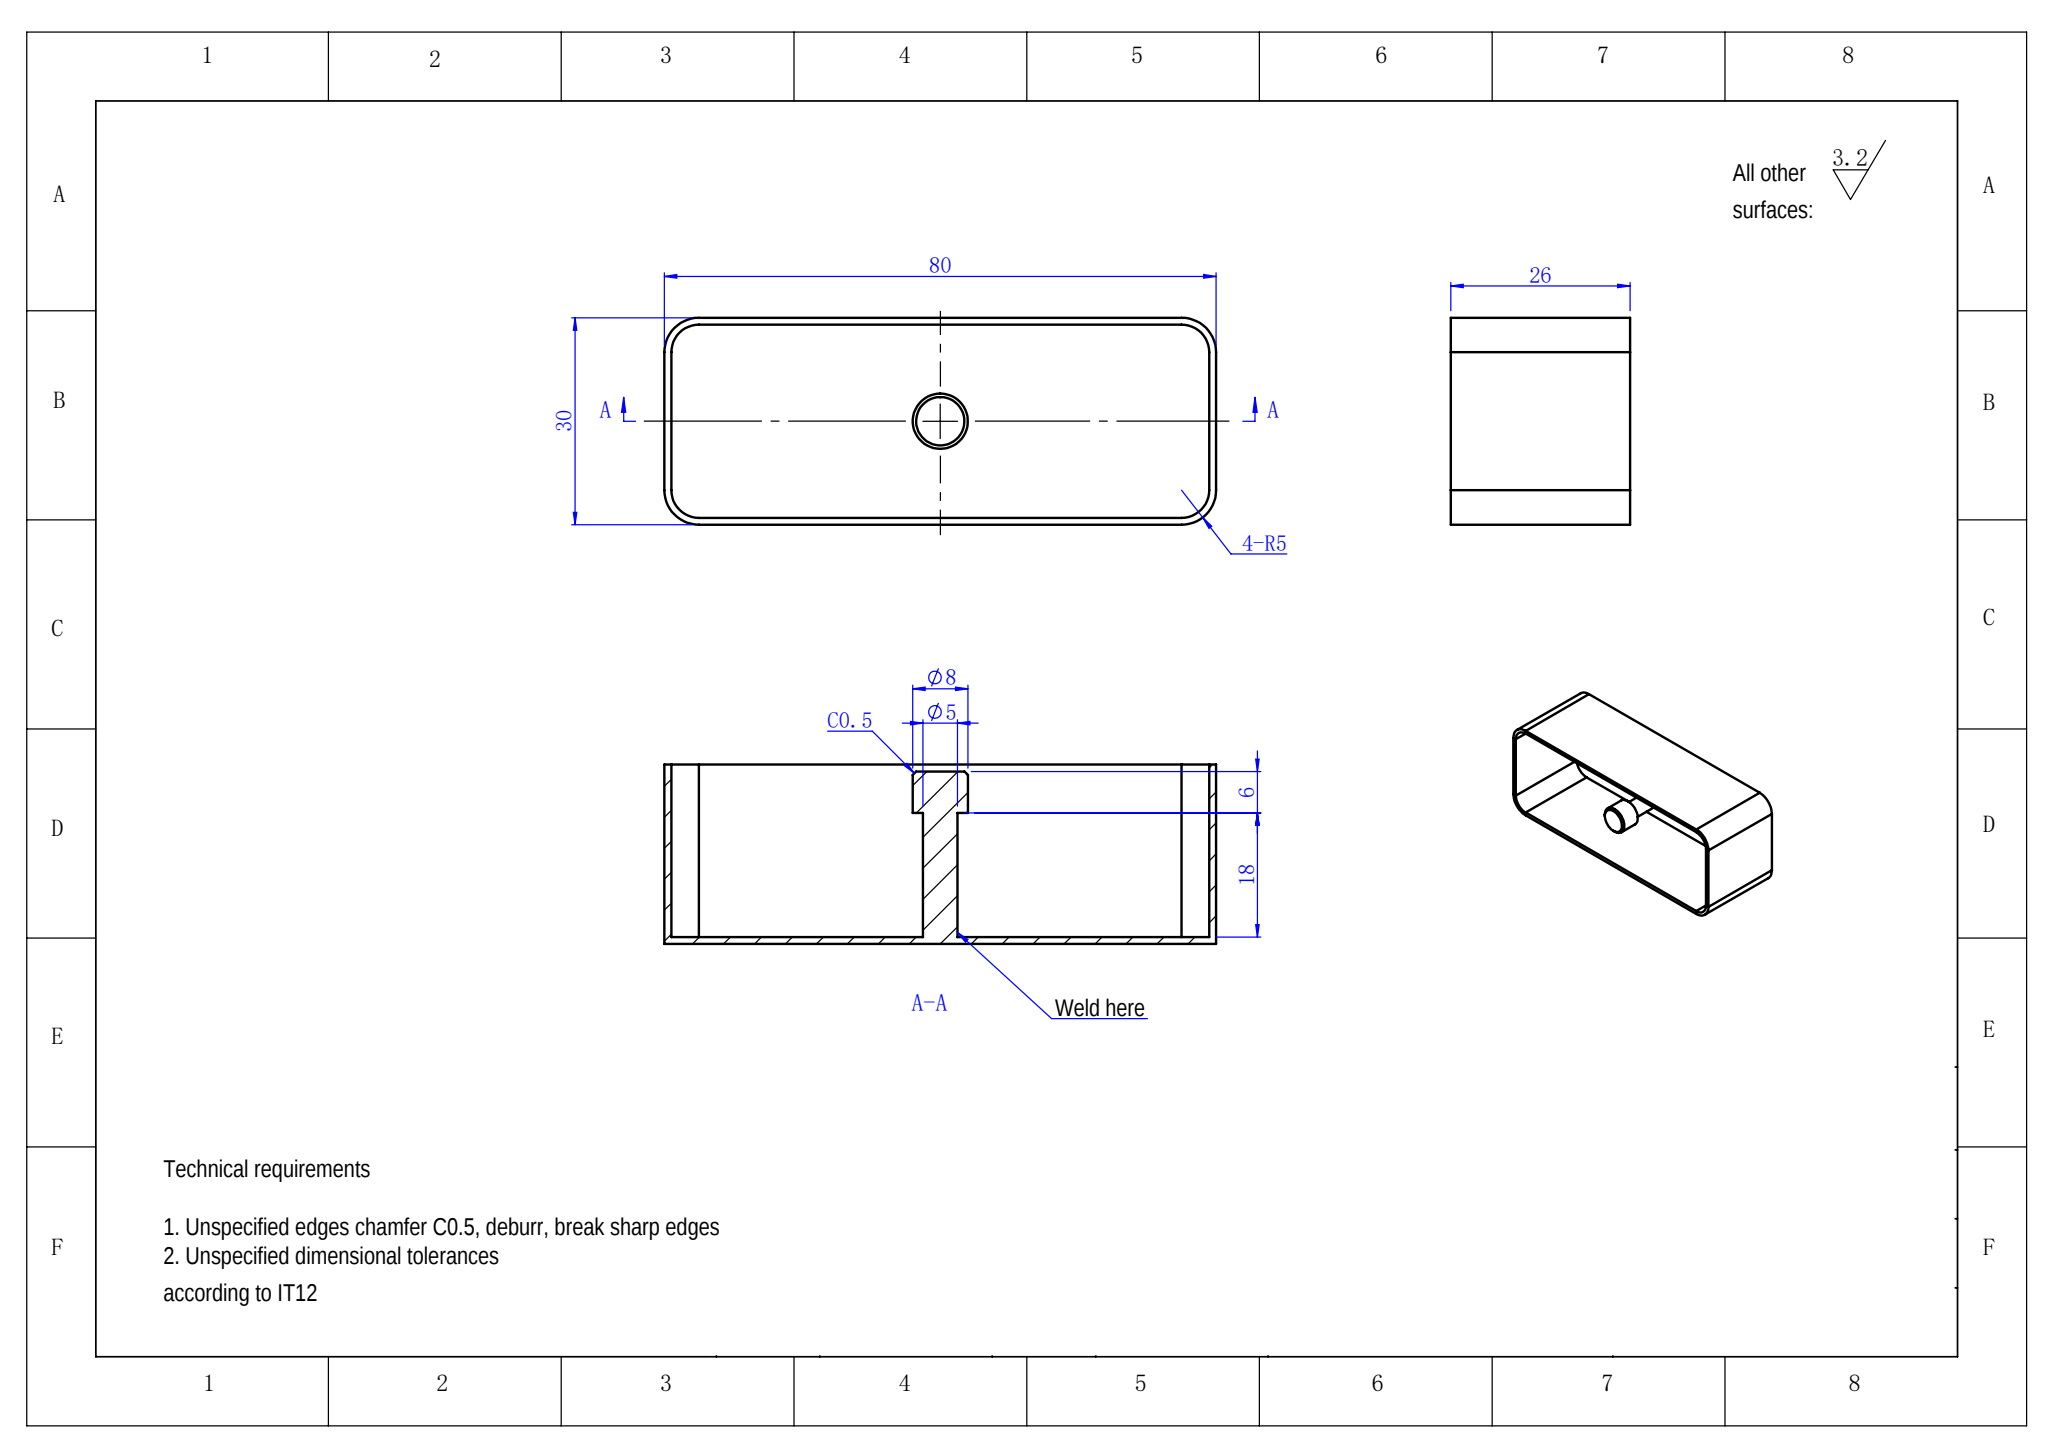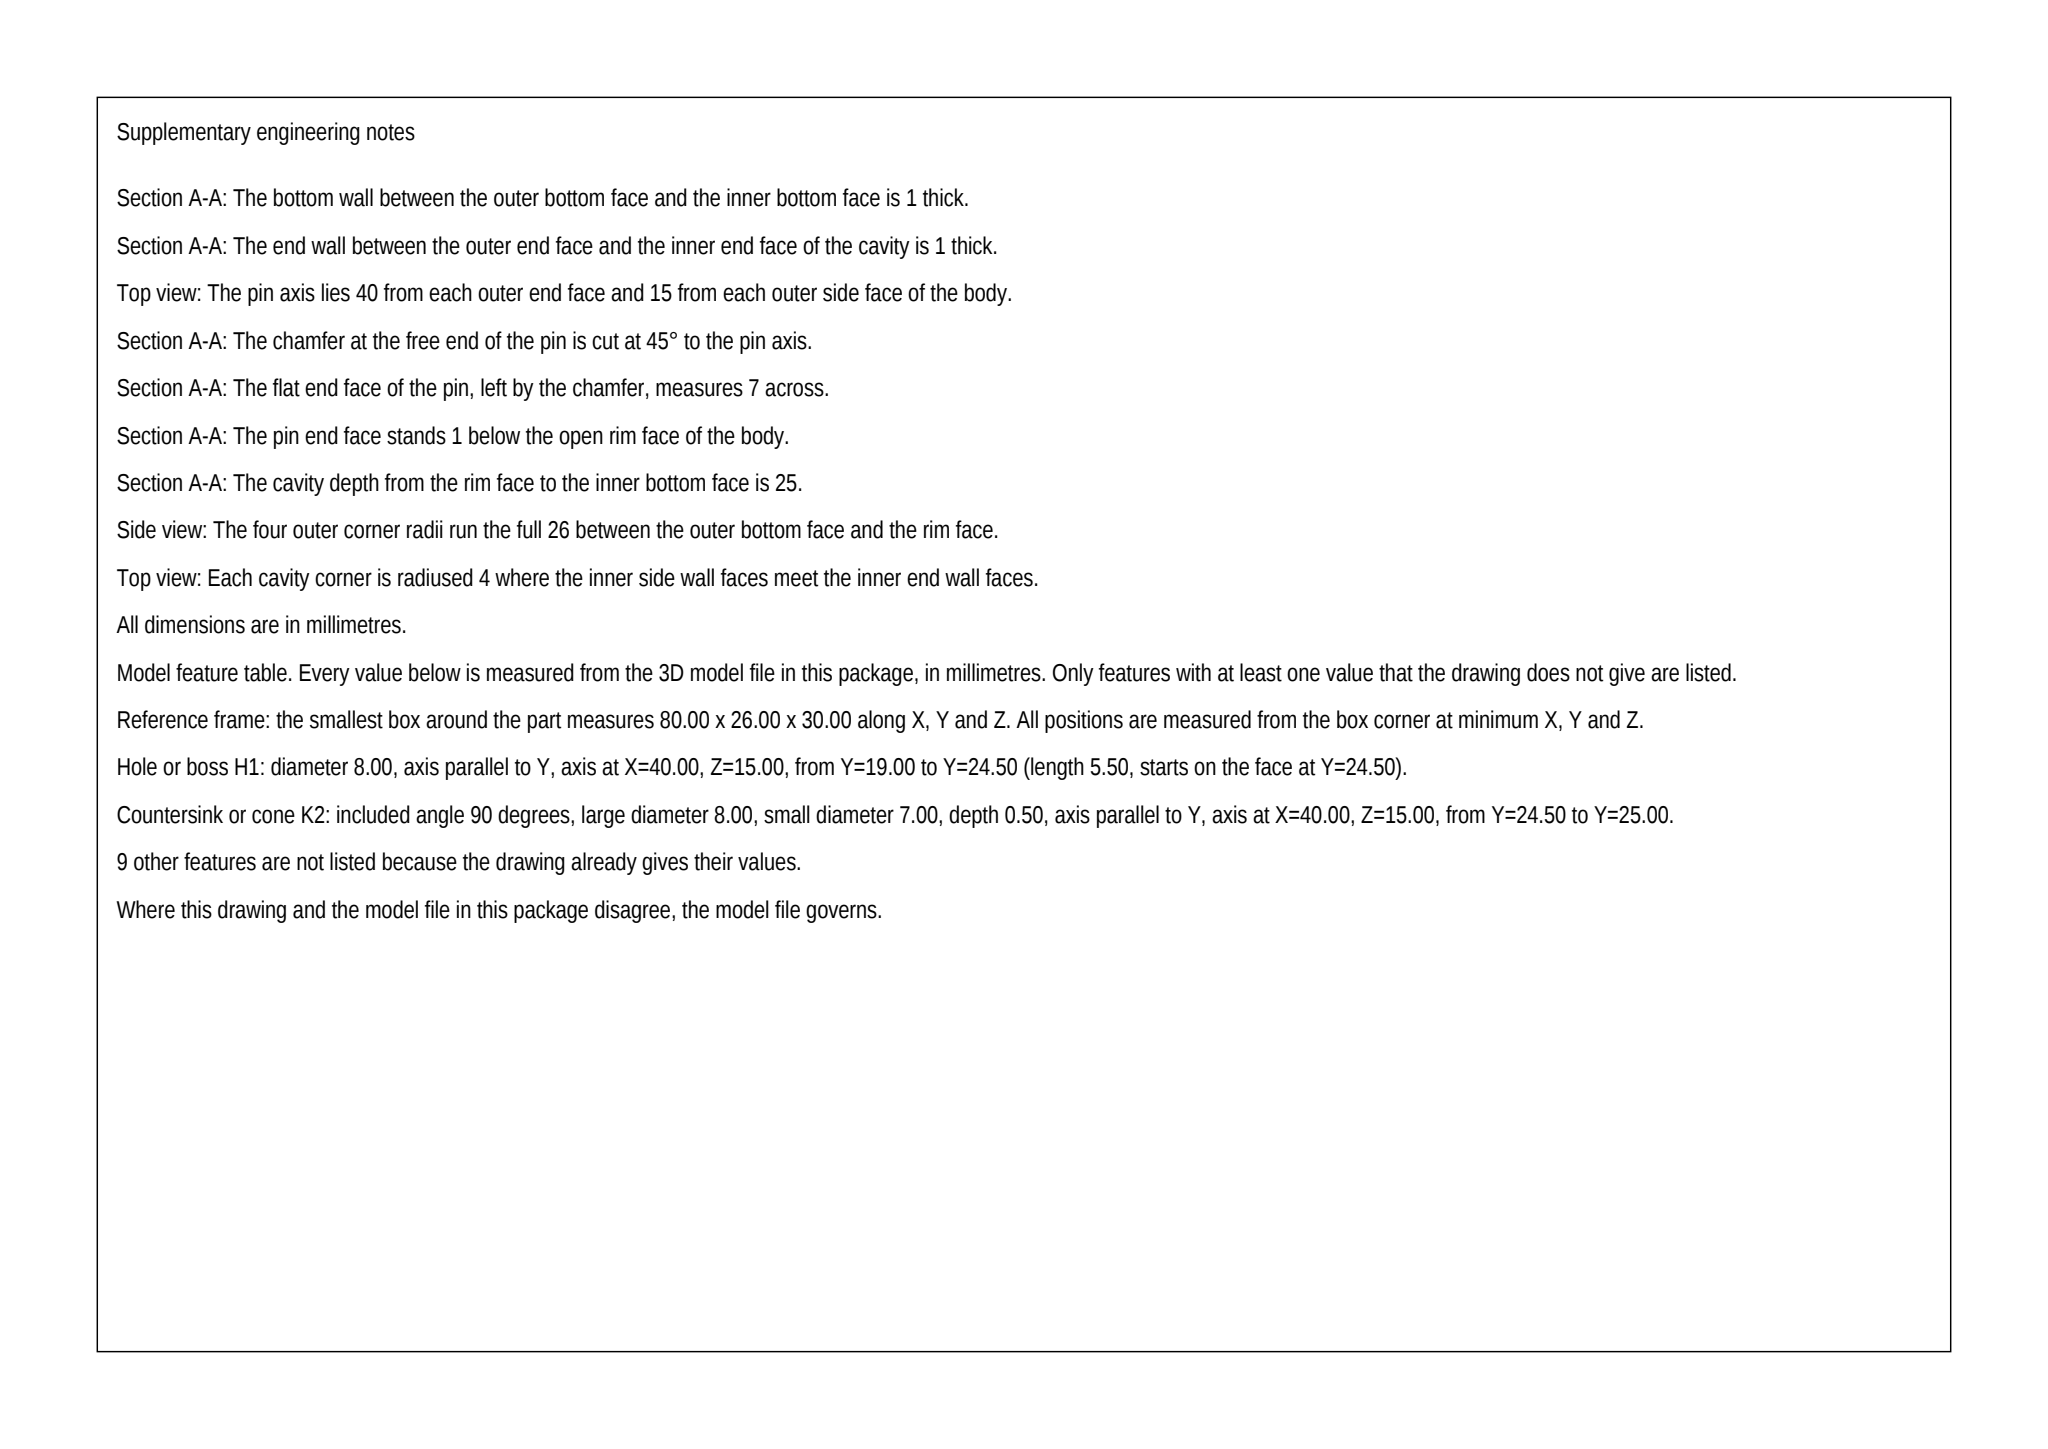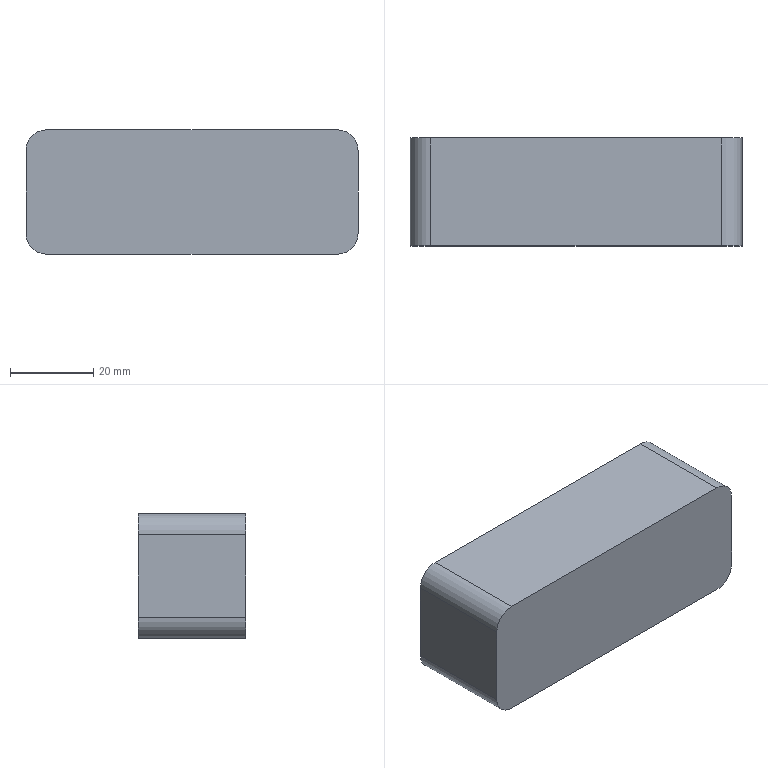Part | SolidWorks | mm | 1 solid | 27 faces | box 80 x 26 x 30 mm | volume 8237 mm3 | plane 13 | cylinder 12 | cone 2 | commonest cylinder face diameters 8 x6 10 x4 5 x2
build123d program:
from build123d import *

# Parameters (mm, degrees)
BOSS_EXTRUDE1_DEPTH = 26
SHELL1_T            = -1
CHAMFER1_SIZE       = 0.5


with BuildPart() as part:
    # Sketch1 → Boss-Extrude1 (new body)
    with BuildSketch(Plane(origin=(0, 0, 0), x_dir=(1, 0, 0), z_dir=(0, 1, 0))):
        with BuildLine():
            Line((-35, 15), (35, 15))
            ThreePointArc((35, 15), (38.536, 13.536), (40, 10))
            Line((40, 10), (40, -10))
            ThreePointArc((40, -10), (38.536, -13.536), (35, -15))
            Line((35, -15), (-35, -15))
            ThreePointArc((-35, -15), (-38.536, -13.536), (-40, -10))
            Line((-40, -10), (-40, 10))
            ThreePointArc((-40, 10), (-38.536, 13.536), (-35, 15))
        make_face()
    extrude(amount=BOSS_EXTRUDE1_DEPTH)

    # Shell1
    shell1_openings = [part.faces().sort_by_distance(p)[0] for p in [
        (0, 26, 0),
    ]]
    offset(amount=SHELL1_T, openings=shell1_openings, kind=Kind.INTERSECTION)

    # Sketch3 → Revolve1 (revolve)
    with BuildSketch(Plane.XY, mode=Mode.PRIVATE) as revolve1_sk:
        Polygon((0, 0), (-2.5, 0), (-2.5, 19), (-4, 19), (-4, 25), (0, 25), align=None)
    revolve(revolve1_sk.sketch.rotate(Axis((0, 0, 0), (0, 1, 0)), 270), axis=Axis((0, 0, 0), (0, 1, 0)))

    # Chamfer1
    chamfer1_edges = [part.edges().sort_by_distance(p)[0] for p in [
        (0, 25, 4),
    ]]
    chamfer(chamfer1_edges, length=CHAMFER1_SIZE)


solid = part.part
STEP:
#1=CARTESIAN_POINT('',(0.,25.,3.5));
#2=VERTEX_POINT('',#1);
#3=CARTESIAN_POINT('',(0.,25.,-3.5));
#4=VERTEX_POINT('',#3);
#5=CARTESIAN_POINT('',(0.,25.,0.));
#6=DIRECTION('',(0.,1.,0.));
#7=DIRECTION('',(0.,0.,-1.));
#8=AXIS2_PLACEMENT_3D('',#5,#6,#7);
#9=CIRCLE('',#8,3.5);
#10=EDGE_CURVE('',#2,#4,#9,.T.);
#11=ORIENTED_EDGE('',*,*,#10,.F.);
#12=CARTESIAN_POINT('',(0.,24.5,4.));
#13=VERTEX_POINT('',#12);
#14=CARTESIAN_POINT('',(0.,24.5,4.));
#15=DIRECTION('',(0.,-0.7071,0.7071));
#16=VECTOR('',#15,1000.);
#17=LINE('',#14,#16);
#18=EDGE_CURVE('',#2,#13,#17,.T.);
#19=ORIENTED_EDGE('',*,*,#18,.T.);
#20=CARTESIAN_POINT('',(0.,24.5,-4.));
#21=VERTEX_POINT('',#20);
#22=CARTESIAN_POINT('',(0.,24.5,0.));
#23=DIRECTION('',(0.,-1.,0.));
#24=DIRECTION('',(0.,0.,-1.));
#25=AXIS2_PLACEMENT_3D('',#22,#23,#24);
#26=CIRCLE('',#25,4.);
#27=EDGE_CURVE('',#21,#13,#26,.T.);
#28=ORIENTED_EDGE('',*,*,#27,.F.);
#29=CARTESIAN_POINT('',(0.,24.5,-4.));
#30=DIRECTION('',(0.,-0.7071,-0.7071));
#31=VECTOR('',#30,1000.);
#32=LINE('',#29,#31);
#33=EDGE_CURVE('',#4,#21,#32,.T.);
#34=ORIENTED_EDGE('',*,*,#33,.F.);
#35=EDGE_LOOP('',(#11,#19,#28,#34));
#36=FACE_OUTER_BOUND('',#35,.T.);
#37=CARTESIAN_POINT('',(0.,24.5,0.));
#38=DIRECTION('',(0.,-1.,0.));
#39=DIRECTION('',(0.,0.,-1.));
#40=AXIS2_PLACEMENT_3D('',#37,#38,#39);
#41=CONICAL_SURFACE('',#40,4.,0.7854);
#42=ADVANCED_FACE('',(#36),#41,.T.);
#43=ORIENTED_EDGE('',*,*,#27,.T.);
#44=CARTESIAN_POINT('',(0.,19.,4.));
#45=VERTEX_POINT('',#44);
#46=CARTESIAN_POINT('',(0.,0.,4.));
#47=DIRECTION('',(0.,-1.,0.));
#48=VECTOR('',#47,1000.);
#49=LINE('',#46,#48);
#50=EDGE_CURVE('',#13,#45,#49,.T.);
#51=ORIENTED_EDGE('',*,*,#50,.T.);
#52=CARTESIAN_POINT('',(0.,19.,-4.));
#53=VERTEX_POINT('',#52);
#54=CARTESIAN_POINT('',(0.,19.,0.));
#55=DIRECTION('',(0.,-1.,0.));
#56=DIRECTION('',(0.,0.,-1.));
#57=AXIS2_PLACEMENT_3D('',#54,#55,#56);
#58=CIRCLE('',#57,4.);
#59=EDGE_CURVE('',#53,#45,#58,.T.);
#60=ORIENTED_EDGE('',*,*,#59,.F.);
#61=CARTESIAN_POINT('',(0.,0.,-4.));
#62=DIRECTION('',(0.,-1.,0.));
#63=VECTOR('',#62,1000.);
#64=LINE('',#61,#63);
#65=EDGE_CURVE('',#21,#53,#64,.T.);
#66=ORIENTED_EDGE('',*,*,#65,.F.);
#67=EDGE_LOOP('',(#43,#51,#60,#66));
#68=FACE_OUTER_BOUND('',#67,.T.);
#69=CARTESIAN_POINT('',(0.,0.,0.));
#70=DIRECTION('',(0.,-1.,0.));
#71=DIRECTION('',(0.,0.,-1.));
#72=AXIS2_PLACEMENT_3D('',#69,#70,#71);
#73=CYLINDRICAL_SURFACE('',#72,4.);
#74=ADVANCED_FACE('',(#68),#73,.T.);
#75=CARTESIAN_POINT('',(0.,19.,-2.5));
#76=VERTEX_POINT('',#75);
#77=CARTESIAN_POINT('',(0.,19.,2.5));
#78=VERTEX_POINT('',#77);
#79=CARTESIAN_POINT('',(0.,19.,0.));
#80=DIRECTION('',(0.,-1.,0.));
#81=DIRECTION('',(0.,0.,-1.));
#82=AXIS2_PLACEMENT_3D('',#79,#80,#81);
#83=CIRCLE('',#82,2.5);
#84=EDGE_CURVE('',#76,#78,#83,.T.);
#85=ORIENTED_EDGE('',*,*,#84,.T.);
#86=CARTESIAN_POINT('',(0.,1.,2.5));
#87=VERTEX_POINT('',#86);
#88=CARTESIAN_POINT('',(0.,0.,2.5));
#89=DIRECTION('',(0.,-1.,0.));
#90=VECTOR('',#89,1000.);
#91=LINE('',#88,#90);
#92=EDGE_CURVE('',#78,#87,#91,.T.);
#93=ORIENTED_EDGE('',*,*,#92,.T.);
#94=CARTESIAN_POINT('',(0.,1.,-2.5));
#95=VERTEX_POINT('',#94);
#96=CARTESIAN_POINT('',(0.,1.,0.));
#97=DIRECTION('',(0.,-1.,0.));
#98=DIRECTION('',(0.,0.,1.));
#99=AXIS2_PLACEMENT_3D('',#96,#97,#98);
#100=CIRCLE('',#99,2.5);
#101=EDGE_CURVE('',#95,#87,#100,.T.);
#102=ORIENTED_EDGE('',*,*,#101,.F.);
#103=CARTESIAN_POINT('',(0.,0.,-2.5));
#104=DIRECTION('',(0.,-1.,0.));
#105=VECTOR('',#104,1000.);
#106=LINE('',#103,#105);
#107=EDGE_CURVE('',#76,#95,#106,.T.);
#108=ORIENTED_EDGE('',*,*,#107,.F.);
#109=EDGE_LOOP('',(#85,#93,#102,#108));
#110=FACE_OUTER_BOUND('',#109,.T.);
#111=CARTESIAN_POINT('',(0.,0.,0.));
#112=DIRECTION('',(0.,-1.,0.));
#113=DIRECTION('',(0.,0.,-1.));
#114=AXIS2_PLACEMENT_3D('',#111,#112,#113);
#115=CYLINDRICAL_SURFACE('',#114,2.5);
#116=ADVANCED_FACE('',(#110),#115,.T.);
#117=CARTESIAN_POINT('',(35.,0.,15.));
#118=VERTEX_POINT('',#117);
#119=CARTESIAN_POINT('',(40.,0.,10.));
#120=VERTEX_POINT('',#119);
#121=CARTESIAN_POINT('',(35.,0.,10.));
#122=DIRECTION('',(0.,1.,0.));
#123=DIRECTION('',(0.,0.,1.));
#124=AXIS2_PLACEMENT_3D('',#121,#122,#123);
#125=CIRCLE('',#124,5.);
#126=EDGE_CURVE('',#118,#120,#125,.T.);
#127=ORIENTED_EDGE('',*,*,#126,.T.);
#128=CARTESIAN_POINT('',(40.,26.,10.));
#129=VERTEX_POINT('',#128);
#130=CARTESIAN_POINT('',(40.,26.,10.));
#131=DIRECTION('',(0.,-1.,0.));
#132=VECTOR('',#131,1000.);
#133=LINE('',#130,#132);
#134=EDGE_CURVE('',#129,#120,#133,.T.);
#135=ORIENTED_EDGE('',*,*,#134,.F.);
#136=CARTESIAN_POINT('',(35.,26.,15.));
#137=VERTEX_POINT('',#136);
#138=CARTESIAN_POINT('',(35.,26.,10.));
#139=DIRECTION('',(0.,1.,0.));
#140=DIRECTION('',(0.,0.,1.));
#141=AXIS2_PLACEMENT_3D('',#138,#139,#140);
#142=CIRCLE('',#141,5.);
#143=EDGE_CURVE('',#137,#129,#142,.T.);
#144=ORIENTED_EDGE('',*,*,#143,.F.);
#145=CARTESIAN_POINT('',(35.,26.,15.));
#146=DIRECTION('',(0.,-1.,0.));
#147=VECTOR('',#146,1000.);
#148=LINE('',#145,#147);
#149=EDGE_CURVE('',#137,#118,#148,.T.);
#150=ORIENTED_EDGE('',*,*,#149,.T.);
#151=EDGE_LOOP('',(#127,#135,#144,#150));
#152=FACE_OUTER_BOUND('',#151,.T.);
#153=CARTESIAN_POINT('',(35.,26.,10.));
#154=DIRECTION('',(0.,-1.,0.));
#155=DIRECTION('',(0.,0.,-1.));
#156=AXIS2_PLACEMENT_3D('',#153,#154,#155);
#157=CYLINDRICAL_SURFACE('',#156,5.);
#158=ADVANCED_FACE('',(#152),#157,.T.);
#159=CARTESIAN_POINT('',(40.,0.,-10.));
#160=VERTEX_POINT('',#159);
#161=CARTESIAN_POINT('',(40.,0.,-10.));
#162=DIRECTION('',(0.,0.,-1.));
#163=VECTOR('',#162,1000.);
#164=LINE('',#161,#163);
#165=EDGE_CURVE('',#120,#160,#164,.T.);
#166=ORIENTED_EDGE('',*,*,#165,.T.);
#167=CARTESIAN_POINT('',(40.,26.,-10.));
#168=VERTEX_POINT('',#167);
#169=CARTESIAN_POINT('',(40.,26.,-10.));
#170=DIRECTION('',(0.,-1.,0.));
#171=VECTOR('',#170,1000.);
#172=LINE('',#169,#171);
#173=EDGE_CURVE('',#168,#160,#172,.T.);
#174=ORIENTED_EDGE('',*,*,#173,.F.);
#175=CARTESIAN_POINT('',(40.,26.,-10.));
#176=DIRECTION('',(0.,0.,-1.));
#177=VECTOR('',#176,1000.);
#178=LINE('',#175,#177);
#179=EDGE_CURVE('',#129,#168,#178,.T.);
#180=ORIENTED_EDGE('',*,*,#179,.F.);
#181=ORIENTED_EDGE('',*,*,#134,.T.);
#182=EDGE_LOOP('',(#166,#174,#180,#181));
#183=FACE_OUTER_BOUND('',#182,.T.);
#184=CARTESIAN_POINT('',(40.,26.,-10.));
#185=DIRECTION('',(-1.,0.,0.));
#186=DIRECTION('',(0.,0.,1.));
#187=AXIS2_PLACEMENT_3D('',#184,#185,#186);
#188=PLANE('',#187);
#189=ADVANCED_FACE('',(#183),#188,.F.);
#190=CARTESIAN_POINT('',(35.,0.,-15.));
#191=VERTEX_POINT('',#190);
#192=CARTESIAN_POINT('',(35.,0.,-10.));
#193=DIRECTION('',(0.,1.,0.));
#194=DIRECTION('',(0.,0.,1.));
#195=AXIS2_PLACEMENT_3D('',#192,#193,#194);
#196=CIRCLE('',#195,5.);
#197=EDGE_CURVE('',#160,#191,#196,.T.);
#198=ORIENTED_EDGE('',*,*,#197,.T.);
#199=CARTESIAN_POINT('',(35.,26.,-15.));
#200=VERTEX_POINT('',#199);
#201=CARTESIAN_POINT('',(35.,26.,-15.));
#202=DIRECTION('',(0.,-1.,0.));
#203=VECTOR('',#202,1000.);
#204=LINE('',#201,#203);
#205=EDGE_CURVE('',#200,#191,#204,.T.);
#206=ORIENTED_EDGE('',*,*,#205,.F.);
#207=CARTESIAN_POINT('',(35.,26.,-10.));
#208=DIRECTION('',(0.,1.,0.));
#209=DIRECTION('',(0.,0.,1.));
#210=AXIS2_PLACEMENT_3D('',#207,#208,#209);
#211=CIRCLE('',#210,5.);
#212=EDGE_CURVE('',#168,#200,#211,.T.);
#213=ORIENTED_EDGE('',*,*,#212,.F.);
#214=ORIENTED_EDGE('',*,*,#173,.T.);
#215=EDGE_LOOP('',(#198,#206,#213,#214));
#216=FACE_OUTER_BOUND('',#215,.T.);
#217=CARTESIAN_POINT('',(35.,26.,-10.));
#218=DIRECTION('',(0.,-1.,0.));
#219=DIRECTION('',(0.,0.,-1.));
#220=AXIS2_PLACEMENT_3D('',#217,#218,#219);
#221=CYLINDRICAL_SURFACE('',#220,5.);
#222=ADVANCED_FACE('',(#216),#221,.T.);
#223=CARTESIAN_POINT('',(-35.,0.,-15.));
#224=VERTEX_POINT('',#223);
#225=CARTESIAN_POINT('',(-35.,0.,-15.));
#226=DIRECTION('',(-1.,0.,-0.));
#227=VECTOR('',#226,1000.);
#228=LINE('',#225,#227);
#229=EDGE_CURVE('',#191,#224,#228,.T.);
#230=ORIENTED_EDGE('',*,*,#229,.T.);
#231=CARTESIAN_POINT('',(-35.,26.,-15.));
#232=VERTEX_POINT('',#231);
#233=CARTESIAN_POINT('',(-35.,26.,-15.));
#234=DIRECTION('',(0.,-1.,0.));
#235=VECTOR('',#234,1000.);
#236=LINE('',#233,#235);
#237=EDGE_CURVE('',#232,#224,#236,.T.);
#238=ORIENTED_EDGE('',*,*,#237,.F.);
#239=CARTESIAN_POINT('',(-35.,26.,-15.));
#240=DIRECTION('',(-1.,0.,-0.));
#241=VECTOR('',#240,1000.);
#242=LINE('',#239,#241);
#243=EDGE_CURVE('',#200,#232,#242,.T.);
#244=ORIENTED_EDGE('',*,*,#243,.F.);
#245=ORIENTED_EDGE('',*,*,#205,.T.);
#246=EDGE_LOOP('',(#230,#238,#244,#245));
#247=FACE_OUTER_BOUND('',#246,.T.);
#248=CARTESIAN_POINT('',(-35.,26.,-15.));
#249=DIRECTION('',(-0.,0.,1.));
#250=DIRECTION('',(1.,0.,0.));
#251=AXIS2_PLACEMENT_3D('',#248,#249,#250);
#252=PLANE('',#251);
#253=ADVANCED_FACE('',(#247),#252,.F.);
#254=CARTESIAN_POINT('',(-40.,0.,-10.));
#255=VERTEX_POINT('',#254);
#256=CARTESIAN_POINT('',(-35.,0.,-10.));
#257=DIRECTION('',(0.,1.,0.));
#258=DIRECTION('',(0.,0.,1.));
#259=AXIS2_PLACEMENT_3D('',#256,#257,#258);
#260=CIRCLE('',#259,5.);
#261=EDGE_CURVE('',#224,#255,#260,.T.);
#262=ORIENTED_EDGE('',*,*,#261,.T.);
#263=CARTESIAN_POINT('',(-40.,26.,-10.));
#264=VERTEX_POINT('',#263);
#265=CARTESIAN_POINT('',(-40.,26.,-10.));
#266=DIRECTION('',(0.,-1.,0.));
#267=VECTOR('',#266,1000.);
#268=LINE('',#265,#267);
#269=EDGE_CURVE('',#264,#255,#268,.T.);
#270=ORIENTED_EDGE('',*,*,#269,.F.);
#271=CARTESIAN_POINT('',(-35.,26.,-10.));
#272=DIRECTION('',(0.,1.,0.));
#273=DIRECTION('',(0.,0.,1.));
#274=AXIS2_PLACEMENT_3D('',#271,#272,#273);
#275=CIRCLE('',#274,5.);
#276=EDGE_CURVE('',#232,#264,#275,.T.);
#277=ORIENTED_EDGE('',*,*,#276,.F.);
#278=ORIENTED_EDGE('',*,*,#237,.T.);
#279=EDGE_LOOP('',(#262,#270,#277,#278));
#280=FACE_OUTER_BOUND('',#279,.T.);
#281=CARTESIAN_POINT('',(-35.,26.,-10.));
#282=DIRECTION('',(0.,-1.,0.));
#283=DIRECTION('',(0.,0.,-1.));
#284=AXIS2_PLACEMENT_3D('',#281,#282,#283);
#285=CYLINDRICAL_SURFACE('',#284,5.);
#286=ADVANCED_FACE('',(#280),#285,.T.);
#287=CARTESIAN_POINT('',(-40.,0.,10.));
#288=VERTEX_POINT('',#287);
#289=CARTESIAN_POINT('',(-40.,0.,-10.));
#290=DIRECTION('',(0.,0.,1.));
#291=VECTOR('',#290,1000.);
#292=LINE('',#289,#291);
#293=EDGE_CURVE('',#255,#288,#292,.T.);
#294=ORIENTED_EDGE('',*,*,#293,.T.);
#295=CARTESIAN_POINT('',(-40.,26.,10.));
#296=VERTEX_POINT('',#295);
#297=CARTESIAN_POINT('',(-40.,26.,10.));
#298=DIRECTION('',(0.,-1.,0.));
#299=VECTOR('',#298,1000.);
#300=LINE('',#297,#299);
#301=EDGE_CURVE('',#296,#288,#300,.T.);
#302=ORIENTED_EDGE('',*,*,#301,.F.);
#303=CARTESIAN_POINT('',(-40.,26.,-10.));
#304=DIRECTION('',(0.,0.,1.));
#305=VECTOR('',#304,1000.);
#306=LINE('',#303,#305);
#307=EDGE_CURVE('',#264,#296,#306,.T.);
#308=ORIENTED_EDGE('',*,*,#307,.F.);
#309=ORIENTED_EDGE('',*,*,#269,.T.);
#310=EDGE_LOOP('',(#294,#302,#308,#309));
#311=FACE_OUTER_BOUND('',#310,.T.);
#312=CARTESIAN_POINT('',(-40.,26.,-10.));
#313=DIRECTION('',(1.,0.,0.));
#314=DIRECTION('',(0.,0.,-1.));
#315=AXIS2_PLACEMENT_3D('',#312,#313,#314);
#316=PLANE('',#315);
#317=ADVANCED_FACE('',(#311),#316,.F.);
#318=CARTESIAN_POINT('',(-35.,0.,15.));
#319=VERTEX_POINT('',#318);
#320=CARTESIAN_POINT('',(-35.,0.,10.));
#321=DIRECTION('',(0.,1.,0.));
#322=DIRECTION('',(0.,0.,1.));
#323=AXIS2_PLACEMENT_3D('',#320,#321,#322);
#324=CIRCLE('',#323,5.);
#325=EDGE_CURVE('',#288,#319,#324,.T.);
#326=ORIENTED_EDGE('',*,*,#325,.T.);
#327=CARTESIAN_POINT('',(-35.,26.,15.));
#328=VERTEX_POINT('',#327);
#329=CARTESIAN_POINT('',(-35.,26.,15.));
#330=DIRECTION('',(0.,-1.,0.));
#331=VECTOR('',#330,1000.);
#332=LINE('',#329,#331);
#333=EDGE_CURVE('',#328,#319,#332,.T.);
#334=ORIENTED_EDGE('',*,*,#333,.F.);
#335=CARTESIAN_POINT('',(-35.,26.,10.));
#336=DIRECTION('',(0.,1.,0.));
#337=DIRECTION('',(0.,0.,1.));
#338=AXIS2_PLACEMENT_3D('',#335,#336,#337);
#339=CIRCLE('',#338,5.);
#340=EDGE_CURVE('',#296,#328,#339,.T.);
#341=ORIENTED_EDGE('',*,*,#340,.F.);
#342=ORIENTED_EDGE('',*,*,#301,.T.);
#343=EDGE_LOOP('',(#326,#334,#341,#342));
#344=FACE_OUTER_BOUND('',#343,.T.);
#345=CARTESIAN_POINT('',(-35.,26.,10.));
#346=DIRECTION('',(0.,-1.,0.));
#347=DIRECTION('',(0.,0.,-1.));
#348=AXIS2_PLACEMENT_3D('',#345,#346,#347);
#349=CYLINDRICAL_SURFACE('',#348,5.);
#350=ADVANCED_FACE('',(#344),#349,.T.);
#351=CARTESIAN_POINT('',(-35.,0.,15.));
#352=DIRECTION('',(1.,0.,0.));
#353=VECTOR('',#352,1000.);
#354=LINE('',#351,#353);
#355=EDGE_CURVE('',#319,#118,#354,.T.);
#356=ORIENTED_EDGE('',*,*,#355,.T.);
#357=ORIENTED_EDGE('',*,*,#149,.F.);
#358=CARTESIAN_POINT('',(-35.,26.,15.));
#359=DIRECTION('',(1.,0.,0.));
#360=VECTOR('',#359,1000.);
#361=LINE('',#358,#360);
#362=EDGE_CURVE('',#328,#137,#361,.T.);
#363=ORIENTED_EDGE('',*,*,#362,.F.);
#364=ORIENTED_EDGE('',*,*,#333,.T.);
#365=EDGE_LOOP('',(#356,#357,#363,#364));
#366=FACE_OUTER_BOUND('',#365,.T.);
#367=CARTESIAN_POINT('',(-35.,26.,15.));
#368=DIRECTION('',(0.,0.,-1.));
#369=DIRECTION('',(-1.,0.,0.));
#370=AXIS2_PLACEMENT_3D('',#367,#368,#369);
#371=PLANE('',#370);
#372=ADVANCED_FACE('',(#366),#371,.F.);
#373=CARTESIAN_POINT('',(35.,26.,14.));
#374=VERTEX_POINT('',#373);
#375=CARTESIAN_POINT('',(39.,26.,10.));
#376=VERTEX_POINT('',#375);
#377=CARTESIAN_POINT('',(35.,26.,10.));
#378=DIRECTION('',(0.,1.,0.));
#379=DIRECTION('',(0.,0.,1.));
#380=AXIS2_PLACEMENT_3D('',#377,#378,#379);
#381=CIRCLE('',#380,4.);
#382=EDGE_CURVE('',#374,#376,#381,.T.);
#383=ORIENTED_EDGE('',*,*,#382,.F.);
#384=CARTESIAN_POINT('',(-35.,26.,14.));
#385=VERTEX_POINT('',#384);
#386=CARTESIAN_POINT('',(-35.,26.,14.));
#387=DIRECTION('',(1.,0.,0.));
#388=VECTOR('',#387,1000.);
#389=LINE('',#386,#388);
#390=EDGE_CURVE('',#385,#374,#389,.T.);
#391=ORIENTED_EDGE('',*,*,#390,.F.);
#392=CARTESIAN_POINT('',(-39.,26.,10.));
#393=VERTEX_POINT('',#392);
#394=CARTESIAN_POINT('',(-35.,26.,10.));
#395=DIRECTION('',(0.,1.,0.));
#396=DIRECTION('',(0.,0.,1.));
#397=AXIS2_PLACEMENT_3D('',#394,#395,#396);
#398=CIRCLE('',#397,4.);
#399=EDGE_CURVE('',#393,#385,#398,.T.);
#400=ORIENTED_EDGE('',*,*,#399,.F.);
#401=CARTESIAN_POINT('',(-39.,26.,-10.));
#402=VERTEX_POINT('',#401);
#403=CARTESIAN_POINT('',(-39.,26.,-10.));
#404=DIRECTION('',(0.,0.,1.));
#405=VECTOR('',#404,1000.);
#406=LINE('',#403,#405);
#407=EDGE_CURVE('',#402,#393,#406,.T.);
#408=ORIENTED_EDGE('',*,*,#407,.F.);
#409=CARTESIAN_POINT('',(-35.,26.,-14.));
#410=VERTEX_POINT('',#409);
#411=CARTESIAN_POINT('',(-35.,26.,-10.));
#412=DIRECTION('',(0.,1.,0.));
#413=DIRECTION('',(0.,0.,1.));
#414=AXIS2_PLACEMENT_3D('',#411,#412,#413);
#415=CIRCLE('',#414,4.);
#416=EDGE_CURVE('',#410,#402,#415,.T.);
#417=ORIENTED_EDGE('',*,*,#416,.F.);
#418=CARTESIAN_POINT('',(35.,26.,-14.));
#419=VERTEX_POINT('',#418);
#420=CARTESIAN_POINT('',(-35.,26.,-14.));
#421=DIRECTION('',(-1.,0.,-0.));
#422=VECTOR('',#421,1000.);
#423=LINE('',#420,#422);
#424=EDGE_CURVE('',#419,#410,#423,.T.);
#425=ORIENTED_EDGE('',*,*,#424,.F.);
#426=CARTESIAN_POINT('',(39.,26.,-10.));
#427=VERTEX_POINT('',#426);
#428=CARTESIAN_POINT('',(35.,26.,-10.));
#429=DIRECTION('',(0.,1.,0.));
#430=DIRECTION('',(0.,0.,1.));
#431=AXIS2_PLACEMENT_3D('',#428,#429,#430);
#432=CIRCLE('',#431,4.);
#433=EDGE_CURVE('',#427,#419,#432,.T.);
#434=ORIENTED_EDGE('',*,*,#433,.F.);
#435=CARTESIAN_POINT('',(39.,26.,-10.));
#436=DIRECTION('',(0.,0.,-1.));
#437=VECTOR('',#436,1000.);
#438=LINE('',#435,#437);
#439=EDGE_CURVE('',#376,#427,#438,.T.);
#440=ORIENTED_EDGE('',*,*,#439,.F.);
#441=EDGE_LOOP('',(#383,#391,#400,#408,#417,#425,#434,#440));
#442=FACE_BOUND('',#441,.T.);
#443=ORIENTED_EDGE('',*,*,#143,.T.);
#444=ORIENTED_EDGE('',*,*,#179,.T.);
#445=ORIENTED_EDGE('',*,*,#212,.T.);
#446=ORIENTED_EDGE('',*,*,#243,.T.);
#447=ORIENTED_EDGE('',*,*,#276,.T.);
#448=ORIENTED_EDGE('',*,*,#307,.T.);
#449=ORIENTED_EDGE('',*,*,#340,.T.);
#450=ORIENTED_EDGE('',*,*,#362,.T.);
#451=EDGE_LOOP('',(#443,#444,#445,#446,#447,#448,#449,#450));
#452=FACE_OUTER_BOUND('',#451,.T.);
#453=CARTESIAN_POINT('',(35.,26.,10.));
#454=DIRECTION('',(0.,1.,0.));
#455=DIRECTION('',(0.,0.,1.));
#456=AXIS2_PLACEMENT_3D('',#453,#454,#455);
#457=PLANE('',#456);
#458=ADVANCED_FACE('',(#442,#452),#457,.T.);
#459=ORIENTED_EDGE('',*,*,#126,.F.);
#460=ORIENTED_EDGE('',*,*,#355,.F.);
#461=ORIENTED_EDGE('',*,*,#325,.F.);
#462=ORIENTED_EDGE('',*,*,#293,.F.);
#463=ORIENTED_EDGE('',*,*,#261,.F.);
#464=ORIENTED_EDGE('',*,*,#229,.F.);
#465=ORIENTED_EDGE('',*,*,#197,.F.);
#466=ORIENTED_EDGE('',*,*,#165,.F.);
#467=EDGE_LOOP('',(#459,#460,#461,#462,#463,#464,#465,#466));
#468=FACE_OUTER_BOUND('',#467,.T.);
#469=CARTESIAN_POINT('',(35.,0.,10.));
#470=DIRECTION('',(0.,1.,0.));
#471=DIRECTION('',(0.,0.,1.));
#472=AXIS2_PLACEMENT_3D('',#469,#470,#471);
#473=PLANE('',#472);
#474=ADVANCED_FACE('',(#468),#473,.F.);
#475=CARTESIAN_POINT('',(35.,1.,14.));
#476=VERTEX_POINT('',#475);
#477=CARTESIAN_POINT('',(39.,1.,10.));
#478=VERTEX_POINT('',#477);
#479=CARTESIAN_POINT('',(35.,1.,10.));
#480=DIRECTION('',(0.,1.,0.));
#481=DIRECTION('',(0.,0.,1.));
#482=AXIS2_PLACEMENT_3D('',#479,#480,#481);
#483=CIRCLE('',#482,4.);
#484=EDGE_CURVE('',#476,#478,#483,.T.);
#485=ORIENTED_EDGE('',*,*,#484,.F.);
#486=CARTESIAN_POINT('',(35.,26.,14.));
#487=DIRECTION('',(0.,-1.,0.));
#488=VECTOR('',#487,1000.);
#489=LINE('',#486,#488);
#490=EDGE_CURVE('',#374,#476,#489,.T.);
#491=ORIENTED_EDGE('',*,*,#490,.F.);
#492=ORIENTED_EDGE('',*,*,#382,.T.);
#493=CARTESIAN_POINT('',(39.,26.,10.));
#494=DIRECTION('',(0.,-1.,0.));
#495=VECTOR('',#494,1000.);
#496=LINE('',#493,#495);
#497=EDGE_CURVE('',#376,#478,#496,.T.);
#498=ORIENTED_EDGE('',*,*,#497,.T.);
#499=EDGE_LOOP('',(#485,#491,#492,#498));
#500=FACE_OUTER_BOUND('',#499,.T.);
#501=CARTESIAN_POINT('',(35.,26.,10.));
#502=DIRECTION('',(0.,-1.,0.));
#503=DIRECTION('',(0.,0.,-1.));
#504=AXIS2_PLACEMENT_3D('',#501,#502,#503);
#505=CYLINDRICAL_SURFACE('',#504,4.);
#506=ADVANCED_FACE('',(#500),#505,.F.);
#507=CARTESIAN_POINT('',(39.,1.,-10.));
#508=VERTEX_POINT('',#507);
#509=CARTESIAN_POINT('',(39.,1.,-10.));
#510=DIRECTION('',(0.,0.,-1.));
#511=VECTOR('',#510,1000.);
#512=LINE('',#509,#511);
#513=EDGE_CURVE('',#478,#508,#512,.T.);
#514=ORIENTED_EDGE('',*,*,#513,.F.);
#515=ORIENTED_EDGE('',*,*,#497,.F.);
#516=ORIENTED_EDGE('',*,*,#439,.T.);
#517=CARTESIAN_POINT('',(39.,26.,-10.));
#518=DIRECTION('',(0.,-1.,0.));
#519=VECTOR('',#518,1000.);
#520=LINE('',#517,#519);
#521=EDGE_CURVE('',#427,#508,#520,.T.);
#522=ORIENTED_EDGE('',*,*,#521,.T.);
#523=EDGE_LOOP('',(#514,#515,#516,#522));
#524=FACE_OUTER_BOUND('',#523,.T.);
#525=CARTESIAN_POINT('',(39.,26.,-10.));
#526=DIRECTION('',(-1.,0.,0.));
#527=DIRECTION('',(0.,0.,1.));
#528=AXIS2_PLACEMENT_3D('',#525,#526,#527);
#529=PLANE('',#528);
#530=ADVANCED_FACE('',(#524),#529,.T.);
#531=CARTESIAN_POINT('',(35.,1.,-14.));
#532=VERTEX_POINT('',#531);
#533=CARTESIAN_POINT('',(35.,1.,-10.));
#534=DIRECTION('',(0.,1.,0.));
#535=DIRECTION('',(0.,0.,1.));
#536=AXIS2_PLACEMENT_3D('',#533,#534,#535);
#537=CIRCLE('',#536,4.);
#538=EDGE_CURVE('',#508,#532,#537,.T.);
#539=ORIENTED_EDGE('',*,*,#538,.F.);
#540=ORIENTED_EDGE('',*,*,#521,.F.);
#541=ORIENTED_EDGE('',*,*,#433,.T.);
#542=CARTESIAN_POINT('',(35.,26.,-14.));
#543=DIRECTION('',(0.,-1.,0.));
#544=VECTOR('',#543,1000.);
#545=LINE('',#542,#544);
#546=EDGE_CURVE('',#419,#532,#545,.T.);
#547=ORIENTED_EDGE('',*,*,#546,.T.);
#548=EDGE_LOOP('',(#539,#540,#541,#547));
#549=FACE_OUTER_BOUND('',#548,.T.);
#550=CARTESIAN_POINT('',(35.,26.,-10.));
#551=DIRECTION('',(0.,-1.,0.));
#552=DIRECTION('',(0.,0.,-1.));
#553=AXIS2_PLACEMENT_3D('',#550,#551,#552);
#554=CYLINDRICAL_SURFACE('',#553,4.);
#555=ADVANCED_FACE('',(#549),#554,.F.);
#556=CARTESIAN_POINT('',(-35.,1.,-14.));
#557=VERTEX_POINT('',#556);
#558=CARTESIAN_POINT('',(-35.,1.,-14.));
#559=DIRECTION('',(-1.,0.,-0.));
#560=VECTOR('',#559,1000.);
#561=LINE('',#558,#560);
#562=EDGE_CURVE('',#532,#557,#561,.T.);
#563=ORIENTED_EDGE('',*,*,#562,.F.);
#564=ORIENTED_EDGE('',*,*,#546,.F.);
#565=ORIENTED_EDGE('',*,*,#424,.T.);
#566=CARTESIAN_POINT('',(-35.,26.,-14.));
#567=DIRECTION('',(0.,-1.,0.));
#568=VECTOR('',#567,1000.);
#569=LINE('',#566,#568);
#570=EDGE_CURVE('',#410,#557,#569,.T.);
#571=ORIENTED_EDGE('',*,*,#570,.T.);
#572=EDGE_LOOP('',(#563,#564,#565,#571));
#573=FACE_OUTER_BOUND('',#572,.T.);
#574=CARTESIAN_POINT('',(-35.,26.,-14.));
#575=DIRECTION('',(-0.,0.,1.));
#576=DIRECTION('',(1.,0.,0.));
#577=AXIS2_PLACEMENT_3D('',#574,#575,#576);
#578=PLANE('',#577);
#579=ADVANCED_FACE('',(#573),#578,.T.);
#580=CARTESIAN_POINT('',(-39.,1.,-10.));
#581=VERTEX_POINT('',#580);
#582=CARTESIAN_POINT('',(-35.,1.,-10.));
#583=DIRECTION('',(0.,1.,0.));
#584=DIRECTION('',(0.,0.,1.));
#585=AXIS2_PLACEMENT_3D('',#582,#583,#584);
#586=CIRCLE('',#585,4.);
#587=EDGE_CURVE('',#557,#581,#586,.T.);
#588=ORIENTED_EDGE('',*,*,#587,.F.);
#589=ORIENTED_EDGE('',*,*,#570,.F.);
#590=ORIENTED_EDGE('',*,*,#416,.T.);
#591=CARTESIAN_POINT('',(-39.,26.,-10.));
#592=DIRECTION('',(0.,-1.,0.));
#593=VECTOR('',#592,1000.);
#594=LINE('',#591,#593);
#595=EDGE_CURVE('',#402,#581,#594,.T.);
#596=ORIENTED_EDGE('',*,*,#595,.T.);
#597=EDGE_LOOP('',(#588,#589,#590,#596));
#598=FACE_OUTER_BOUND('',#597,.T.);
#599=CARTESIAN_POINT('',(-35.,26.,-10.));
#600=DIRECTION('',(0.,-1.,0.));
#601=DIRECTION('',(0.,0.,-1.));
#602=AXIS2_PLACEMENT_3D('',#599,#600,#601);
#603=CYLINDRICAL_SURFACE('',#602,4.);
#604=ADVANCED_FACE('',(#598),#603,.F.);
#605=CARTESIAN_POINT('',(-39.,1.,10.));
#606=VERTEX_POINT('',#605);
#607=CARTESIAN_POINT('',(-39.,1.,-10.));
#608=DIRECTION('',(0.,0.,1.));
#609=VECTOR('',#608,1000.);
#610=LINE('',#607,#609);
#611=EDGE_CURVE('',#581,#606,#610,.T.);
#612=ORIENTED_EDGE('',*,*,#611,.F.);
#613=ORIENTED_EDGE('',*,*,#595,.F.);
#614=ORIENTED_EDGE('',*,*,#407,.T.);
#615=CARTESIAN_POINT('',(-39.,26.,10.));
#616=DIRECTION('',(0.,-1.,0.));
#617=VECTOR('',#616,1000.);
#618=LINE('',#615,#617);
#619=EDGE_CURVE('',#393,#606,#618,.T.);
#620=ORIENTED_EDGE('',*,*,#619,.T.);
#621=EDGE_LOOP('',(#612,#613,#614,#620));
#622=FACE_OUTER_BOUND('',#621,.T.);
#623=CARTESIAN_POINT('',(-39.,26.,-10.));
#624=DIRECTION('',(1.,0.,0.));
#625=DIRECTION('',(0.,0.,-1.));
#626=AXIS2_PLACEMENT_3D('',#623,#624,#625);
#627=PLANE('',#626);
#628=ADVANCED_FACE('',(#622),#627,.T.);
#629=CARTESIAN_POINT('',(-35.,1.,14.));
#630=VERTEX_POINT('',#629);
#631=CARTESIAN_POINT('',(-35.,1.,10.));
#632=DIRECTION('',(0.,1.,0.));
#633=DIRECTION('',(0.,0.,1.));
#634=AXIS2_PLACEMENT_3D('',#631,#632,#633);
#635=CIRCLE('',#634,4.);
#636=EDGE_CURVE('',#606,#630,#635,.T.);
#637=ORIENTED_EDGE('',*,*,#636,.F.);
#638=ORIENTED_EDGE('',*,*,#619,.F.);
#639=ORIENTED_EDGE('',*,*,#399,.T.);
#640=CARTESIAN_POINT('',(-35.,26.,14.));
#641=DIRECTION('',(0.,-1.,0.));
#642=VECTOR('',#641,1000.);
#643=LINE('',#640,#642);
#644=EDGE_CURVE('',#385,#630,#643,.T.);
#645=ORIENTED_EDGE('',*,*,#644,.T.);
#646=EDGE_LOOP('',(#637,#638,#639,#645));
#647=FACE_OUTER_BOUND('',#646,.T.);
#648=CARTESIAN_POINT('',(-35.,26.,10.));
#649=DIRECTION('',(0.,-1.,0.));
#650=DIRECTION('',(0.,0.,-1.));
#651=AXIS2_PLACEMENT_3D('',#648,#649,#650);
#652=CYLINDRICAL_SURFACE('',#651,4.);
#653=ADVANCED_FACE('',(#647),#652,.F.);
#654=CARTESIAN_POINT('',(-35.,1.,14.));
#655=DIRECTION('',(1.,0.,0.));
#656=VECTOR('',#655,1000.);
#657=LINE('',#654,#656);
#658=EDGE_CURVE('',#630,#476,#657,.T.);
#659=ORIENTED_EDGE('',*,*,#658,.F.);
#660=ORIENTED_EDGE('',*,*,#644,.F.);
#661=ORIENTED_EDGE('',*,*,#390,.T.);
#662=ORIENTED_EDGE('',*,*,#490,.T.);
#663=EDGE_LOOP('',(#659,#660,#661,#662));
#664=FACE_OUTER_BOUND('',#663,.T.);
#665=CARTESIAN_POINT('',(-35.,26.,14.));
#666=DIRECTION('',(0.,0.,-1.));
#667=DIRECTION('',(-1.,0.,0.));
#668=AXIS2_PLACEMENT_3D('',#665,#666,#667);
#669=PLANE('',#668);
#670=ADVANCED_FACE('',(#664),#669,.T.);
#671=ORIENTED_EDGE('',*,*,#101,.T.);
#672=CARTESIAN_POINT('',(0.,1.,0.));
#673=DIRECTION('',(0.,-1.,0.));
#674=DIRECTION('',(0.,0.,1.));
#675=AXIS2_PLACEMENT_3D('',#672,#673,#674);
#676=CIRCLE('',#675,2.5);
#677=EDGE_CURVE('',#87,#95,#676,.T.);
#678=ORIENTED_EDGE('',*,*,#677,.T.);
#679=EDGE_LOOP('',(#671,#678));
#680=FACE_BOUND('',#679,.T.);
#681=ORIENTED_EDGE('',*,*,#484,.T.);
#682=ORIENTED_EDGE('',*,*,#513,.T.);
#683=ORIENTED_EDGE('',*,*,#538,.T.);
#684=ORIENTED_EDGE('',*,*,#562,.T.);
#685=ORIENTED_EDGE('',*,*,#587,.T.);
#686=ORIENTED_EDGE('',*,*,#611,.T.);
#687=ORIENTED_EDGE('',*,*,#636,.T.);
#688=ORIENTED_EDGE('',*,*,#658,.T.);
#689=EDGE_LOOP('',(#681,#682,#683,#684,#685,#686,#687,#688));
#690=FACE_OUTER_BOUND('',#689,.T.);
#691=CARTESIAN_POINT('',(35.,1.,10.));
#692=DIRECTION('',(0.,1.,0.));
#693=DIRECTION('',(0.,0.,1.));
#694=AXIS2_PLACEMENT_3D('',#691,#692,#693);
#695=PLANE('',#694);
#696=ADVANCED_FACE('',(#680,#690),#695,.T.);
#697=ORIENTED_EDGE('',*,*,#92,.F.);
#698=CARTESIAN_POINT('',(0.,19.,0.));
#699=DIRECTION('',(0.,-1.,0.));
#700=DIRECTION('',(0.,0.,-1.));
#701=AXIS2_PLACEMENT_3D('',#698,#699,#700);
#702=CIRCLE('',#701,2.5);
#703=EDGE_CURVE('',#78,#76,#702,.T.);
#704=ORIENTED_EDGE('',*,*,#703,.T.);
#705=ORIENTED_EDGE('',*,*,#107,.T.);
#706=ORIENTED_EDGE('',*,*,#677,.F.);
#707=EDGE_LOOP('',(#697,#704,#705,#706));
#708=FACE_OUTER_BOUND('',#707,.T.);
#709=CARTESIAN_POINT('',(0.,0.,0.));
#710=DIRECTION('',(0.,-1.,0.));
#711=DIRECTION('',(0.,0.,-1.));
#712=AXIS2_PLACEMENT_3D('',#709,#710,#711);
#713=CYLINDRICAL_SURFACE('',#712,2.5);
#714=ADVANCED_FACE('',(#708),#713,.T.);
#715=ORIENTED_EDGE('',*,*,#84,.F.);
#716=ORIENTED_EDGE('',*,*,#703,.F.);
#717=EDGE_LOOP('',(#715,#716));
#718=FACE_BOUND('',#717,.T.);
#719=ORIENTED_EDGE('',*,*,#59,.T.);
#720=CARTESIAN_POINT('',(0.,19.,0.));
#721=DIRECTION('',(0.,-1.,0.));
#722=DIRECTION('',(0.,0.,-1.));
#723=AXIS2_PLACEMENT_3D('',#720,#721,#722);
#724=CIRCLE('',#723,4.);
#725=EDGE_CURVE('',#45,#53,#724,.T.);
#726=ORIENTED_EDGE('',*,*,#725,.T.);
#727=EDGE_LOOP('',(#719,#726));
#728=FACE_OUTER_BOUND('',#727,.T.);
#729=CARTESIAN_POINT('',(-2.5,19.,0.));
#730=DIRECTION('',(0.,1.,0.));
#731=DIRECTION('',(0.,0.,1.));
#732=AXIS2_PLACEMENT_3D('',#729,#730,#731);
#733=PLANE('',#732);
#734=ADVANCED_FACE('',(#718,#728),#733,.F.);
#735=ORIENTED_EDGE('',*,*,#50,.F.);
#736=CARTESIAN_POINT('',(0.,24.5,0.));
#737=DIRECTION('',(0.,-1.,0.));
#738=DIRECTION('',(0.,0.,-1.));
#739=AXIS2_PLACEMENT_3D('',#736,#737,#738);
#740=CIRCLE('',#739,4.);
#741=EDGE_CURVE('',#13,#21,#740,.T.);
#742=ORIENTED_EDGE('',*,*,#741,.T.);
#743=ORIENTED_EDGE('',*,*,#65,.T.);
#744=ORIENTED_EDGE('',*,*,#725,.F.);
#745=EDGE_LOOP('',(#735,#742,#743,#744));
#746=FACE_OUTER_BOUND('',#745,.T.);
#747=CARTESIAN_POINT('',(0.,0.,0.));
#748=DIRECTION('',(0.,-1.,0.));
#749=DIRECTION('',(0.,0.,-1.));
#750=AXIS2_PLACEMENT_3D('',#747,#748,#749);
#751=CYLINDRICAL_SURFACE('',#750,4.);
#752=ADVANCED_FACE('',(#746),#751,.T.);
#753=CARTESIAN_POINT('',(0.,25.,0.));
#754=DIRECTION('',(0.,1.,0.));
#755=DIRECTION('',(0.,0.,-1.));
#756=AXIS2_PLACEMENT_3D('',#753,#754,#755);
#757=CIRCLE('',#756,3.5);
#758=EDGE_CURVE('',#4,#2,#757,.T.);
#759=ORIENTED_EDGE('',*,*,#758,.T.);
#760=ORIENTED_EDGE('',*,*,#10,.T.);
#761=EDGE_LOOP('',(#759,#760));
#762=FACE_OUTER_BOUND('',#761,.T.);
#763=CARTESIAN_POINT('',(-4.,25.,0.));
#764=DIRECTION('',(0.,-1.,0.));
#765=DIRECTION('',(0.,0.,-1.));
#766=AXIS2_PLACEMENT_3D('',#763,#764,#765);
#767=PLANE('',#766);
#768=ADVANCED_FACE('',(#762),#767,.F.);
#769=ORIENTED_EDGE('',*,*,#18,.F.);
#770=ORIENTED_EDGE('',*,*,#758,.F.);
#771=ORIENTED_EDGE('',*,*,#33,.T.);
#772=ORIENTED_EDGE('',*,*,#741,.F.);
#773=EDGE_LOOP('',(#769,#770,#771,#772));
#774=FACE_OUTER_BOUND('',#773,.T.);
#775=CARTESIAN_POINT('',(0.,24.5,0.));
#776=DIRECTION('',(0.,-1.,0.));
#777=DIRECTION('',(0.,0.,-1.));
#778=AXIS2_PLACEMENT_3D('',#775,#776,#777);
#779=CONICAL_SURFACE('',#778,4.,0.7854);
#780=ADVANCED_FACE('',(#774),#779,.T.);
#781=CLOSED_SHELL('',(#42,#74,#116,#158,#189,#222,#253,#286,#317,#350,#372,#458,#474,#506,#530,#555,#579,#604,#628,#653,#670,#696,#714,#734,#752,#768,#780));
#782=MANIFOLD_SOLID_BREP('',#781);
#783=CARTESIAN_POINT('',(0.,0.,0.));
#784=DIRECTION('',(0.,0.,1.));
#785=DIRECTION('',(1.,0.,0.));
#786=AXIS2_PLACEMENT_3D('',#783,#784,#785);
#787=(LENGTH_UNIT()NAMED_UNIT(*)SI_UNIT(.MILLI.,.METRE.));
#788=UNCERTAINTY_MEASURE_WITH_UNIT(LENGTH_MEASURE(0.00001),#787,'','');
#789=(NAMED_UNIT(*)PLANE_ANGLE_UNIT()SI_UNIT($,.RADIAN.));
#790=(NAMED_UNIT(*)SI_UNIT($,.STERADIAN.)SOLID_ANGLE_UNIT());
#791=(GEOMETRIC_REPRESENTATION_CONTEXT(3)GLOBAL_UNCERTAINTY_ASSIGNED_CONTEXT((#788))GLOBAL_UNIT_ASSIGNED_CONTEXT((#787,#789,#790))REPRESENTATION_CONTEXT('',''));
#792=ADVANCED_BREP_SHAPE_REPRESENTATION('',(#782,#786),#791);